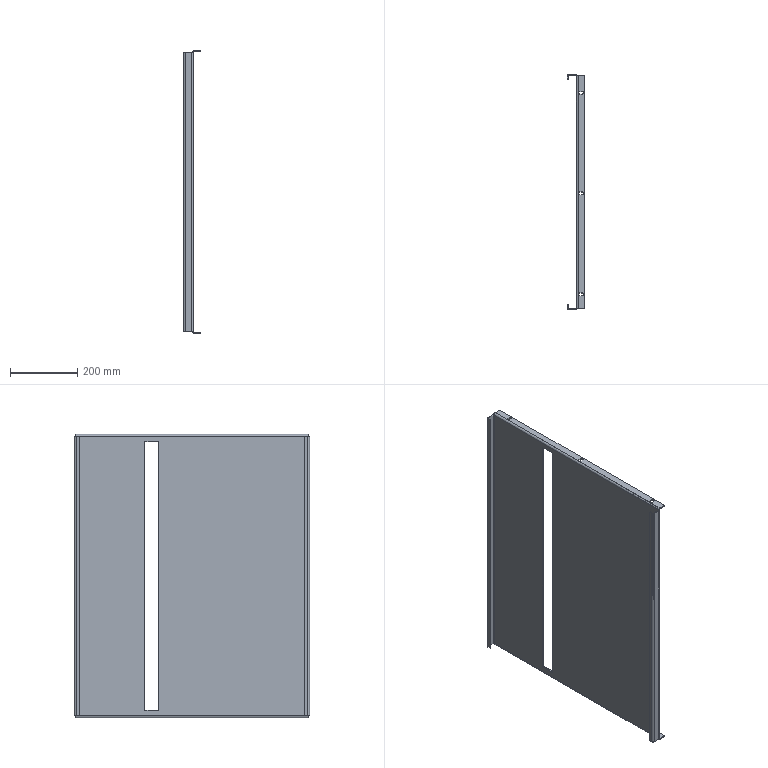Component | SolidWorks | MainMountingPlateF4-00-3 | 1 solid | 92 faces | volume 1931516 mm3 | plane 62 | cylinder 30 | commonest cylinder face diameters 9 x18 11 x6 5 x6